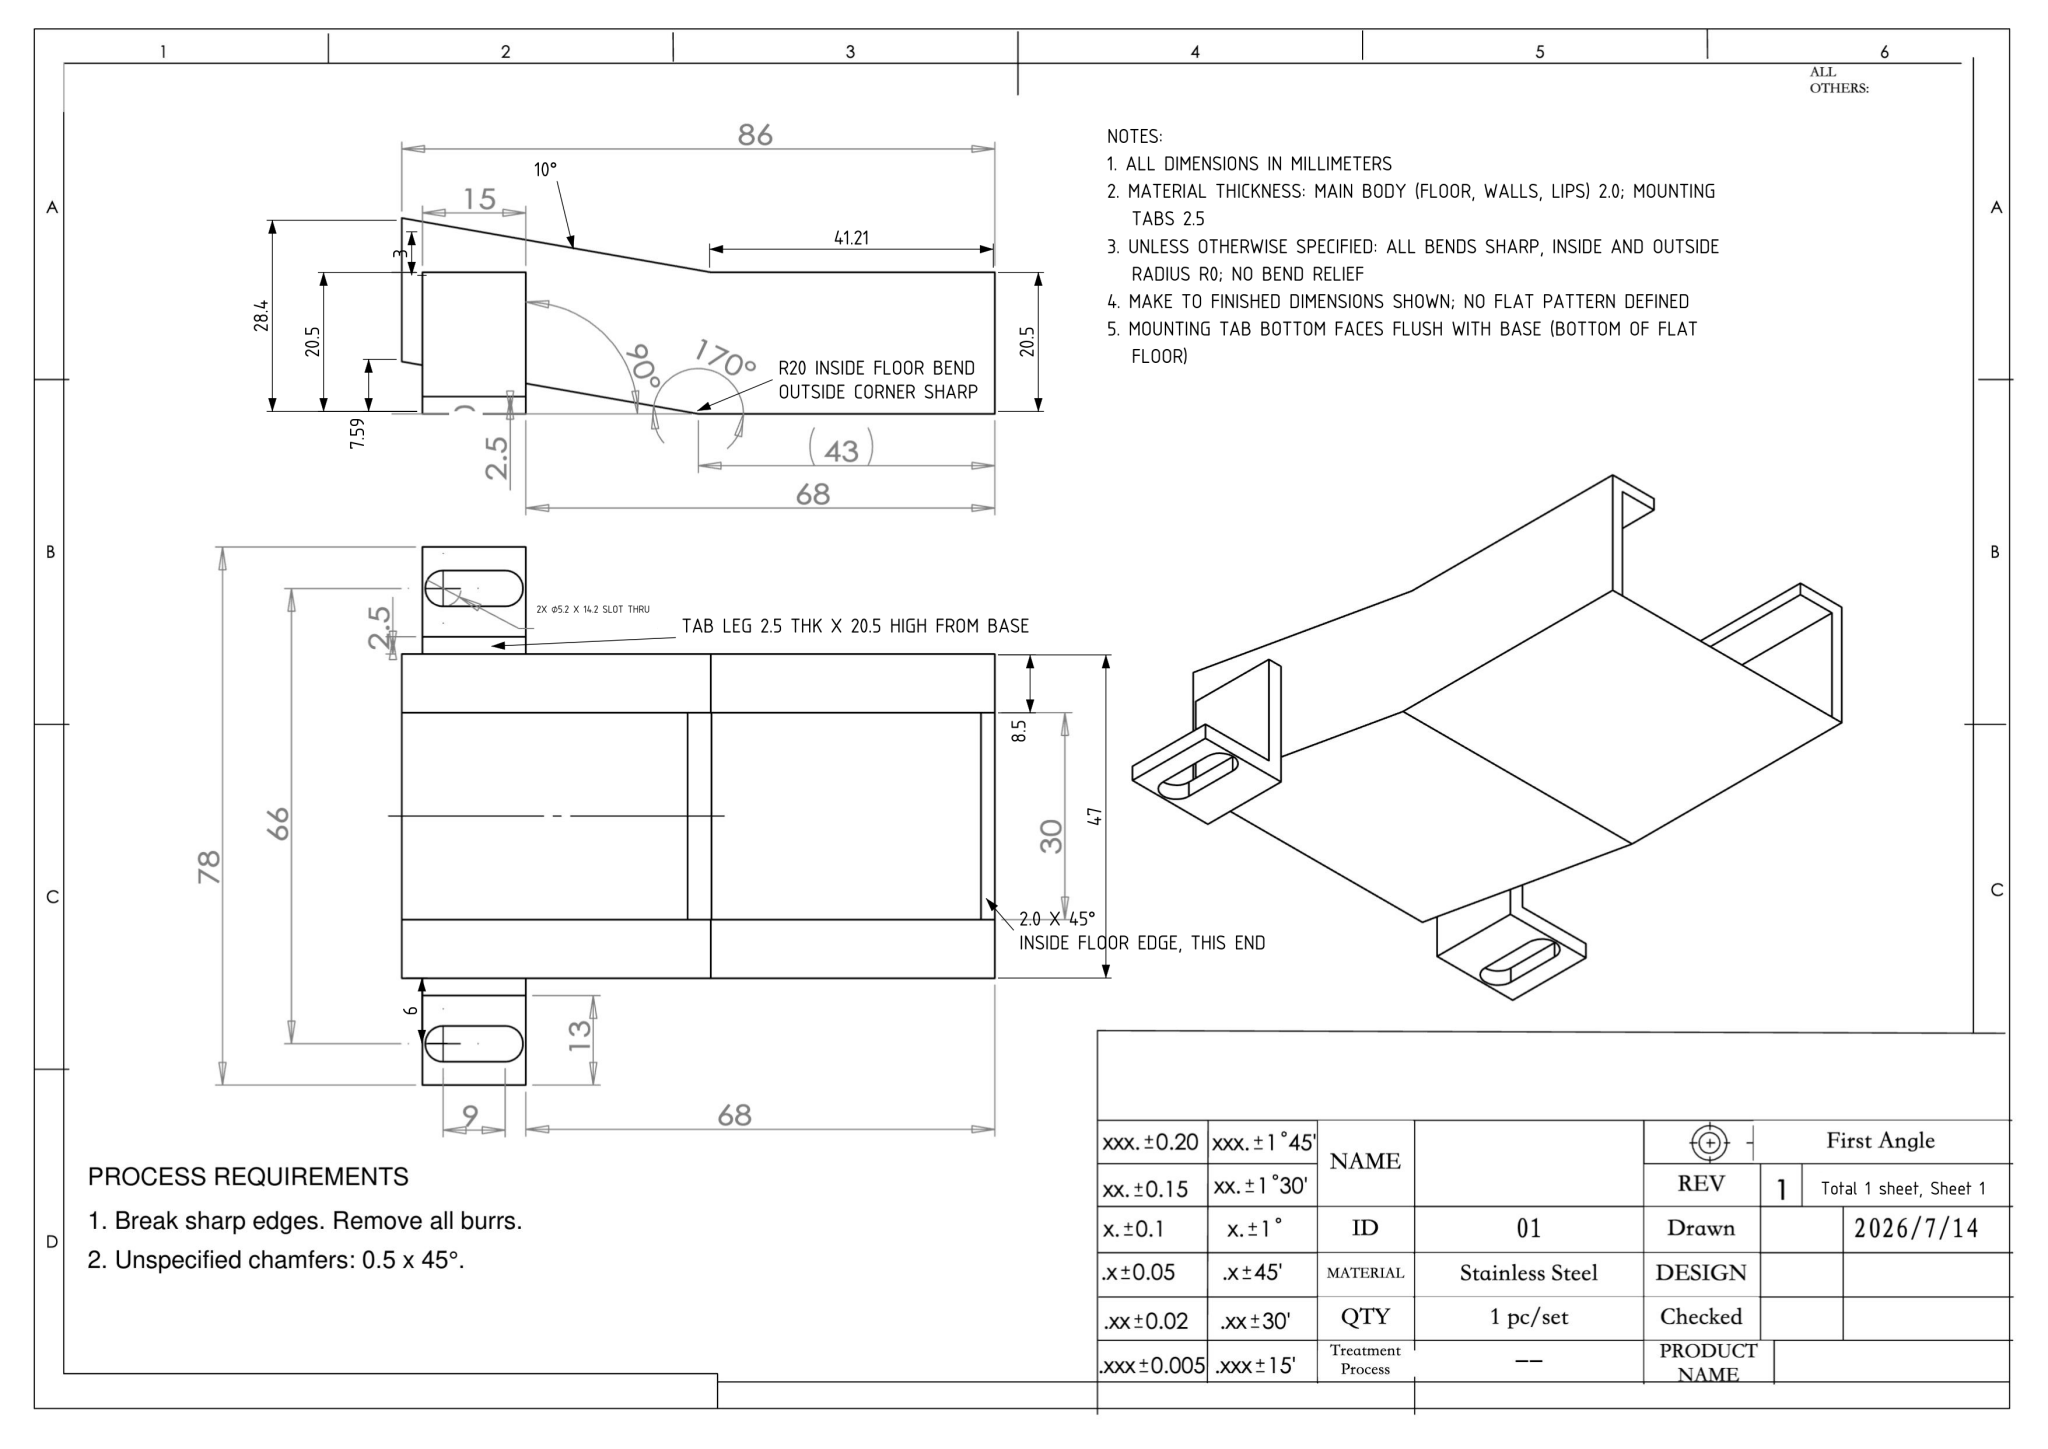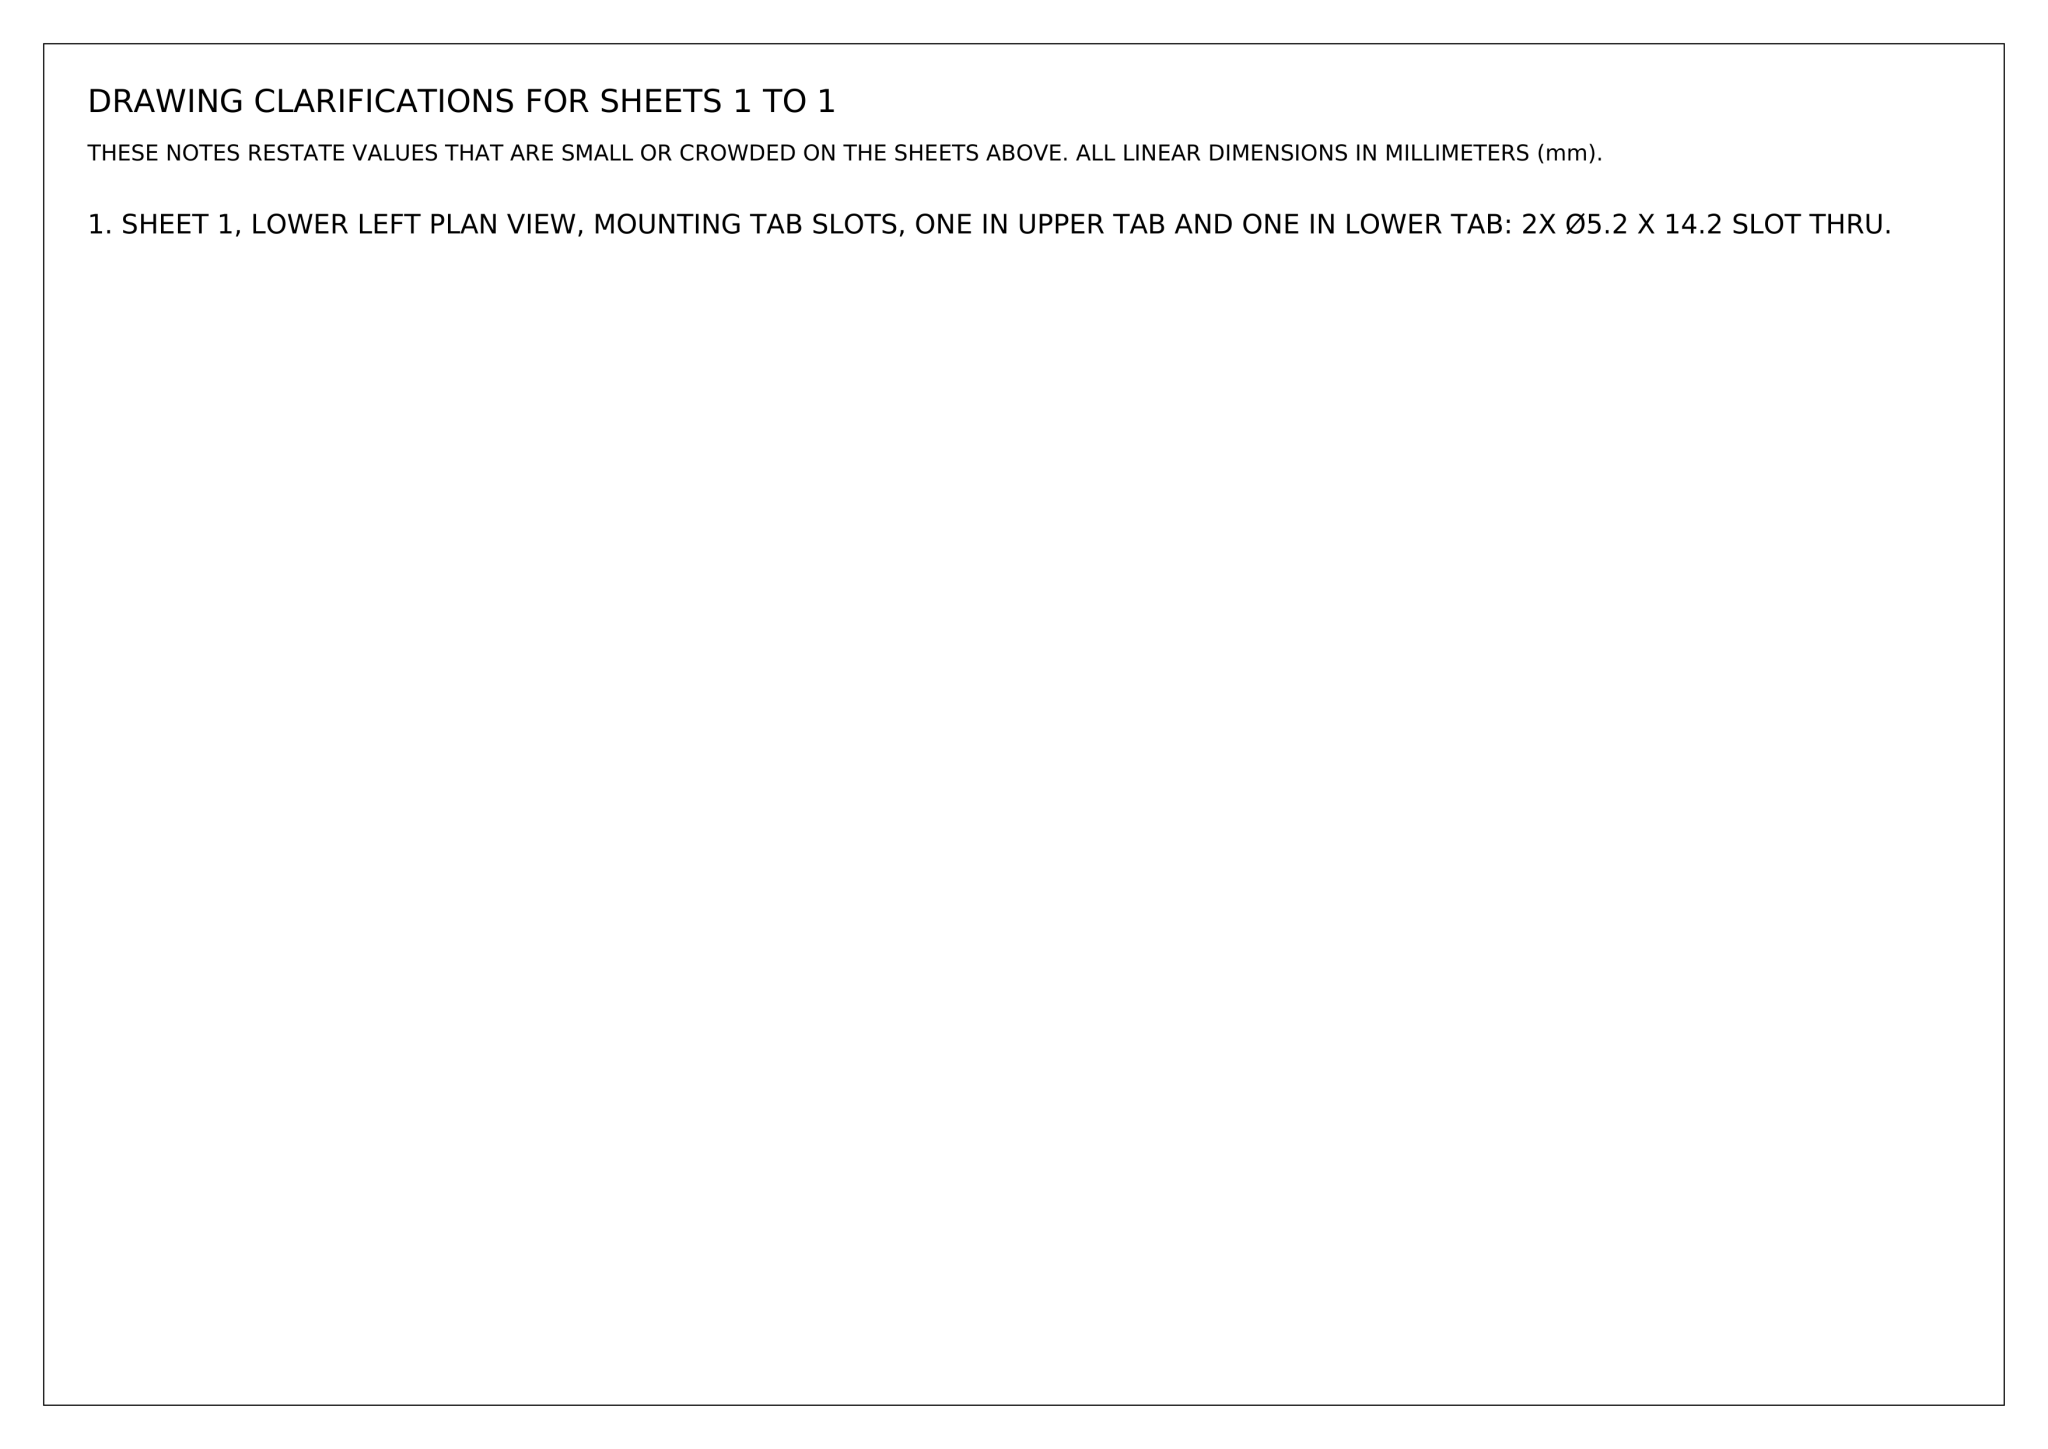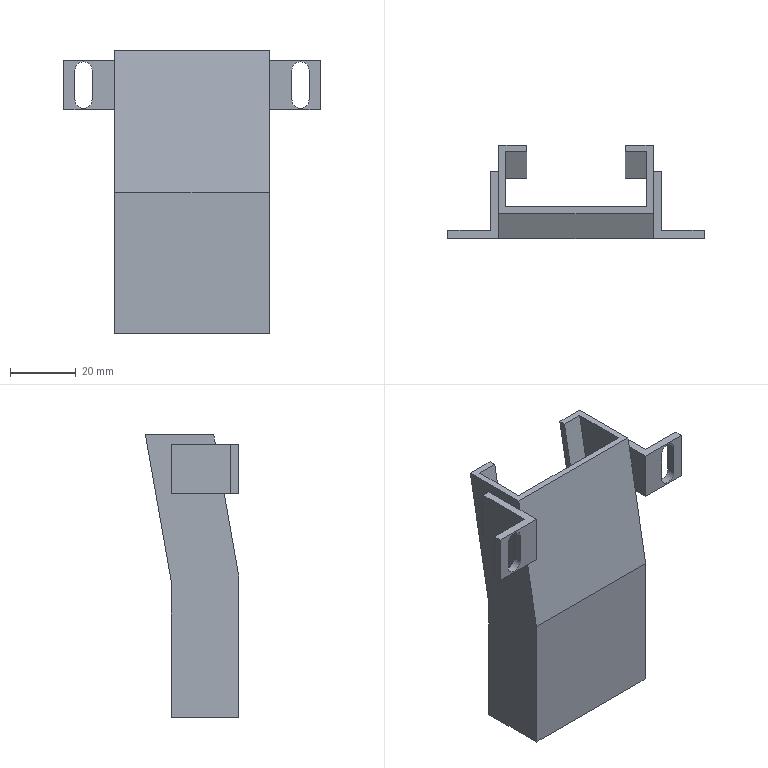Part | NX | mm | Curved Panel Mounting Bracket | 1 solid | 49 faces | box 78 x 28.4 x 86 mm | volume 18905 mm3 | plane 42 | cylinder 7 | commonest cylinder face diameters 5.2 x6 40 x1